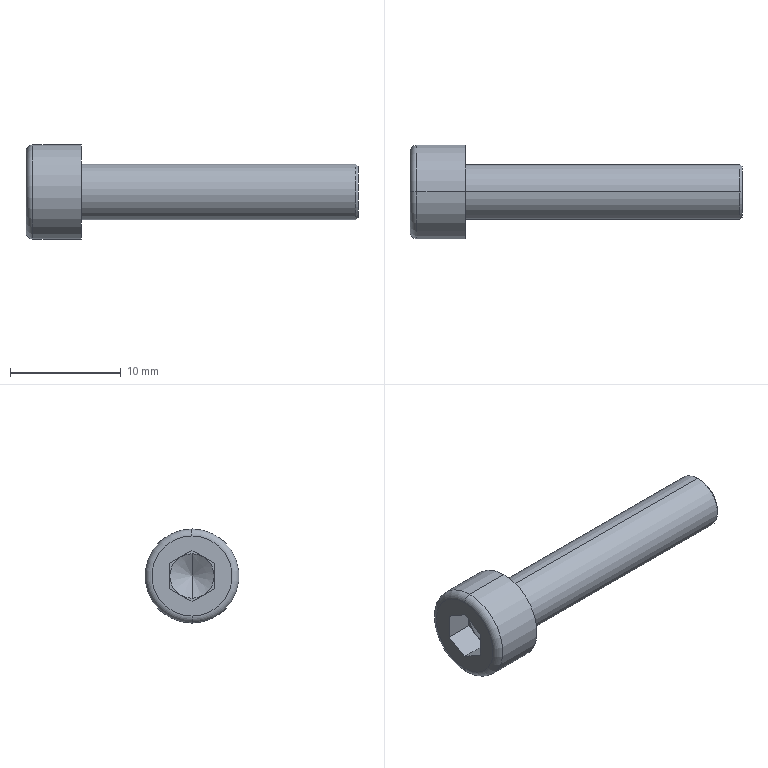Component | SolidWorks | hexagon socket head cap screws gb-26 | 1 solid | 25 faces | volume 733 mm3 | plane 15 | cone 4 | cylinder 4 | torus 2 | commonest cylinder face diameters 5 x2 8.5 x2